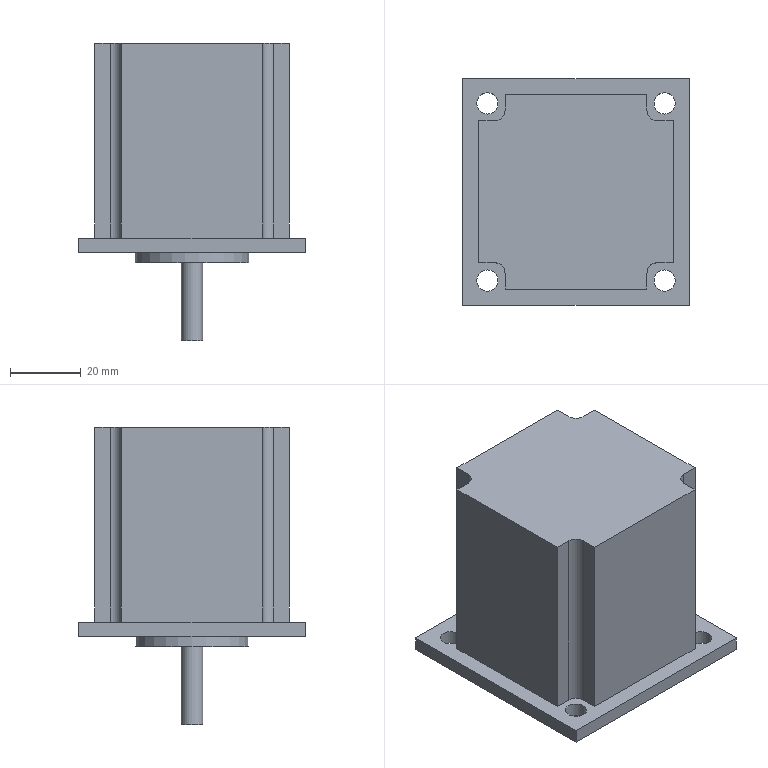Component | NX | MOTOR_1 | 1 solid | 31 faces | volume 173391 mm3 | plane 21 | cylinder 10 | commonest cylinder face diameters 6 x9 32 x1